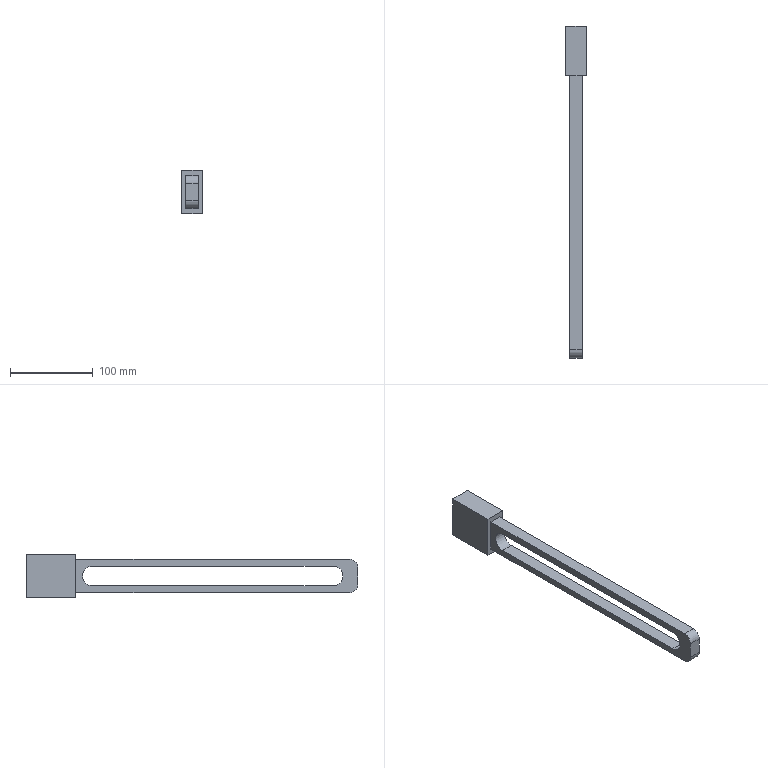Component | SolidWorks | TelescopicRod-1 | 1 solid | 17 faces | box 25 x 400 x 53 mm | volume 171670 mm3 | plane 13 | cylinder 4 | commonest cylinder face diameters 20 x2 24 x2
build123d program:
from build123d import *

# Parameters (mm, degrees)
SKETCH2_W           = 25
SKETCH2_H           = 53
BOSS_EXTRUDE1_DEPTH = 60
SKETCH3_W           = 15
SKETCH3_H           = 40
BOSS_EXTRUDE2_DEPTH = 340
FILLET1_R           = 10
CUT_EXTRUDE1_DEPTH  = 20


with BuildPart() as part:
    # Sketch2 → Boss-Extrude1 (new body)
    with BuildSketch(Plane.XY):
        with Locations((-42.5, 129)):
            Rectangle(SKETCH2_W, SKETCH2_H)
    extrude(amount=BOSS_EXTRUDE1_DEPTH)

    # Sketch3 → Boss-Extrude2 (add)
    with BuildSketch(Plane.XY.offset(60)):
        with Locations((-42.5, 129)):
            Rectangle(SKETCH3_W, SKETCH3_H)
    extrude(amount=BOSS_EXTRUDE2_DEPTH)

    # Fillet1
    fillet1_edges = [part.edges().sort_by_distance(p)[0] for p in [
        (-42.5, 109, 400),
        (-42.5, 149, 400),
    ]]
    fillet(fillet1_edges, radius=FILLET1_R)

    # Sketch4 → Cut-Extrude1 (cut)
    with BuildSketch(Plane.ZY.offset(50)):
        with BuildLine():
            Line((370, 117), (80, 117))
            ThreePointArc((80, 117), (68, 129), (80, 141))
            Line((80, 141), (370, 141))
            ThreePointArc((370, 141), (382, 129), (370, 117))
        make_face()
    extrude(amount=-CUT_EXTRUDE1_DEPTH, mode=Mode.SUBTRACT)


solid = part.part

# Placed as in the assembly
solid = solid.moved(Location((-496.496, 273.496, 244.626), (90, 0, 0)))
STEP:
#1=COLOUR_RGB('',0.7922,0.8196,0.9333);
#2=FILL_AREA_STYLE_COLOUR('',#1);
#3=FILL_AREA_STYLE('',(#2));
#4=SURFACE_STYLE_FILL_AREA(#3);
#5=SURFACE_SIDE_STYLE('',(#4));
#6=SURFACE_STYLE_USAGE(.BOTH.,#5);
#7=PRESENTATION_STYLE_ASSIGNMENT((#6));
#8=CARTESIAN_POINT('',(-21.712,10.768,15.753));
#9=VERTEX_POINT('',#8);
#10=CARTESIAN_POINT('',(-21.712,10.768,13.666));
#11=VERTEX_POINT('',#10);
#12=CARTESIAN_POINT('',(-21.712,10.768,15.753));
#13=DIRECTION('',(-0.,-0.,-1.));
#14=VECTOR('',#13,39.37);
#15=LINE('',#12,#14);
#16=EDGE_CURVE('',#9,#11,#15,.T.);
#17=ORIENTED_EDGE('',*,*,#16,.T.);
#18=CARTESIAN_POINT('',(-21.712,8.405,13.666));
#19=VERTEX_POINT('',#18);
#20=CARTESIAN_POINT('',(-21.712,8.405,13.666));
#21=DIRECTION('',(0.,1.,-0.));
#22=VECTOR('',#21,39.37);
#23=LINE('',#20,#22);
#24=EDGE_CURVE('',#19,#11,#23,.T.);
#25=ORIENTED_EDGE('',*,*,#24,.F.);
#26=CARTESIAN_POINT('',(-21.712,8.405,15.753));
#27=VERTEX_POINT('',#26);
#28=CARTESIAN_POINT('',(-21.712,8.405,15.753));
#29=DIRECTION('',(-0.,-0.,-1.));
#30=VECTOR('',#29,39.37);
#31=LINE('',#28,#30);
#32=EDGE_CURVE('',#27,#19,#31,.T.);
#33=ORIENTED_EDGE('',*,*,#32,.F.);
#34=CARTESIAN_POINT('',(-21.712,8.405,15.753));
#35=DIRECTION('',(0.,1.,-0.));
#36=VECTOR('',#35,39.37);
#37=LINE('',#34,#36);
#38=EDGE_CURVE('',#27,#9,#37,.T.);
#39=ORIENTED_EDGE('',*,*,#38,.T.);
#40=EDGE_LOOP('',(#17,#25,#33,#39));
#41=FACE_OUTER_BOUND('',#40,.T.);
#42=CARTESIAN_POINT('',(-21.712,8.405,15.753));
#43=DIRECTION('',(1.,-0.,-0.));
#44=DIRECTION('',(0.,1.,-0.));
#45=AXIS2_PLACEMENT_3D('',#42,#43,#44);
#46=PLANE('',#45);
#47=ADVANCED_FACE('',(#41),#46,.F.);
#48=CARTESIAN_POINT('',(-20.728,10.768,13.666));
#49=VERTEX_POINT('',#48);
#50=CARTESIAN_POINT('',(-21.712,10.768,13.666));
#51=DIRECTION('',(1.,-0.,0.));
#52=VECTOR('',#51,39.37);
#53=LINE('',#50,#52);
#54=EDGE_CURVE('',#11,#49,#53,.T.);
#55=ORIENTED_EDGE('',*,*,#54,.T.);
#56=CARTESIAN_POINT('',(-20.728,8.405,13.666));
#57=VERTEX_POINT('',#56);
#58=CARTESIAN_POINT('',(-20.728,8.405,13.666));
#59=DIRECTION('',(0.,1.,-0.));
#60=VECTOR('',#59,39.37);
#61=LINE('',#58,#60);
#62=EDGE_CURVE('',#57,#49,#61,.T.);
#63=ORIENTED_EDGE('',*,*,#62,.F.);
#64=CARTESIAN_POINT('',(-21.712,8.405,13.666));
#65=DIRECTION('',(1.,-0.,0.));
#66=VECTOR('',#65,39.37);
#67=LINE('',#64,#66);
#68=EDGE_CURVE('',#19,#57,#67,.T.);
#69=ORIENTED_EDGE('',*,*,#68,.F.);
#70=ORIENTED_EDGE('',*,*,#24,.T.);
#71=EDGE_LOOP('',(#55,#63,#69,#70));
#72=FACE_OUTER_BOUND('',#71,.T.);
#73=CARTESIAN_POINT('',(-21.712,8.405,13.666));
#74=DIRECTION('',(-0.,0.,1.));
#75=DIRECTION('',(-1.,0.,-0.));
#76=AXIS2_PLACEMENT_3D('',#73,#74,#75);
#77=PLANE('',#76);
#78=ADVANCED_FACE('',(#72),#77,.F.);
#79=CARTESIAN_POINT('',(-20.728,10.768,15.753));
#80=VERTEX_POINT('',#79);
#81=CARTESIAN_POINT('',(-20.728,10.768,15.753));
#82=DIRECTION('',(0.,0.,1.));
#83=VECTOR('',#82,39.37);
#84=LINE('',#81,#83);
#85=EDGE_CURVE('',#49,#80,#84,.T.);
#86=ORIENTED_EDGE('',*,*,#85,.T.);
#87=CARTESIAN_POINT('',(-20.728,8.405,15.753));
#88=VERTEX_POINT('',#87);
#89=CARTESIAN_POINT('',(-20.728,8.405,15.753));
#90=DIRECTION('',(0.,1.,-0.));
#91=VECTOR('',#90,39.37);
#92=LINE('',#89,#91);
#93=EDGE_CURVE('',#88,#80,#92,.T.);
#94=ORIENTED_EDGE('',*,*,#93,.F.);
#95=CARTESIAN_POINT('',(-20.728,8.405,15.753));
#96=DIRECTION('',(0.,0.,1.));
#97=VECTOR('',#96,39.37);
#98=LINE('',#95,#97);
#99=EDGE_CURVE('',#57,#88,#98,.T.);
#100=ORIENTED_EDGE('',*,*,#99,.F.);
#101=ORIENTED_EDGE('',*,*,#62,.T.);
#102=EDGE_LOOP('',(#86,#94,#100,#101));
#103=FACE_OUTER_BOUND('',#102,.T.);
#104=CARTESIAN_POINT('',(-20.728,8.405,15.753));
#105=DIRECTION('',(-1.,0.,0.));
#106=DIRECTION('',(-0.,-0.,-1.));
#107=AXIS2_PLACEMENT_3D('',#104,#105,#106);
#108=PLANE('',#107);
#109=ADVANCED_FACE('',(#103),#108,.F.);
#110=CARTESIAN_POINT('',(-21.712,10.768,15.753));
#111=DIRECTION('',(-1.,0.,0.));
#112=VECTOR('',#111,39.37);
#113=LINE('',#110,#112);
#114=EDGE_CURVE('',#80,#9,#113,.T.);
#115=ORIENTED_EDGE('',*,*,#114,.T.);
#116=ORIENTED_EDGE('',*,*,#38,.F.);
#117=CARTESIAN_POINT('',(-21.712,8.405,15.753));
#118=DIRECTION('',(-1.,0.,0.));
#119=VECTOR('',#118,39.37);
#120=LINE('',#117,#119);
#121=EDGE_CURVE('',#88,#27,#120,.T.);
#122=ORIENTED_EDGE('',*,*,#121,.F.);
#123=ORIENTED_EDGE('',*,*,#93,.T.);
#124=EDGE_LOOP('',(#115,#116,#122,#123));
#125=FACE_OUTER_BOUND('',#124,.T.);
#126=CARTESIAN_POINT('',(-21.712,8.405,15.753));
#127=DIRECTION('',(-0.,-0.,-1.));
#128=DIRECTION('',(0.,1.,-0.));
#129=AXIS2_PLACEMENT_3D('',#126,#127,#128);
#130=PLANE('',#129);
#131=ADVANCED_FACE('',(#125),#130,.F.);
#132=CARTESIAN_POINT('',(-21.516,8.405,15.497));
#133=VERTEX_POINT('',#132);
#134=CARTESIAN_POINT('',(-21.516,8.405,13.922));
#135=VERTEX_POINT('',#134);
#136=CARTESIAN_POINT('',(-21.516,8.405,15.497));
#137=DIRECTION('',(0.,-0.,-1.));
#138=VECTOR('',#137,39.37);
#139=LINE('',#136,#138);
#140=EDGE_CURVE('',#133,#135,#139,.T.);
#141=ORIENTED_EDGE('',*,*,#140,.F.);
#142=CARTESIAN_POINT('',(-20.925,8.405,15.497));
#143=VERTEX_POINT('',#142);
#144=CARTESIAN_POINT('',(-21.516,8.405,15.497));
#145=DIRECTION('',(-1.,0.,0.));
#146=VECTOR('',#145,39.37);
#147=LINE('',#144,#146);
#148=EDGE_CURVE('',#143,#133,#147,.T.);
#149=ORIENTED_EDGE('',*,*,#148,.F.);
#150=CARTESIAN_POINT('',(-20.925,8.405,13.922));
#151=VERTEX_POINT('',#150);
#152=CARTESIAN_POINT('',(-20.925,8.405,15.497));
#153=DIRECTION('',(-0.,0.,1.));
#154=VECTOR('',#153,39.37);
#155=LINE('',#152,#154);
#156=EDGE_CURVE('',#151,#143,#155,.T.);
#157=ORIENTED_EDGE('',*,*,#156,.F.);
#158=CARTESIAN_POINT('',(-21.516,8.405,13.922));
#159=DIRECTION('',(1.,-0.,-0.));
#160=VECTOR('',#159,39.37);
#161=LINE('',#158,#160);
#162=EDGE_CURVE('',#135,#151,#161,.T.);
#163=ORIENTED_EDGE('',*,*,#162,.F.);
#164=EDGE_LOOP('',(#141,#149,#157,#163));
#165=FACE_BOUND('',#164,.T.);
#166=ORIENTED_EDGE('',*,*,#32,.T.);
#167=ORIENTED_EDGE('',*,*,#68,.T.);
#168=ORIENTED_EDGE('',*,*,#99,.T.);
#169=ORIENTED_EDGE('',*,*,#121,.T.);
#170=EDGE_LOOP('',(#166,#167,#168,#169));
#171=FACE_OUTER_BOUND('',#170,.T.);
#172=CARTESIAN_POINT('',(-19.547,8.405,9.631));
#173=DIRECTION('',(-0.,-1.,0.));
#174=DIRECTION('',(1.,-0.,-0.));
#175=AXIS2_PLACEMENT_3D('',#172,#173,#174);
#176=PLANE('',#175);
#177=ADVANCED_FACE('',(#165,#171),#176,.T.);
#178=ORIENTED_EDGE('',*,*,#16,.F.);
#179=ORIENTED_EDGE('',*,*,#114,.F.);
#180=ORIENTED_EDGE('',*,*,#85,.F.);
#181=ORIENTED_EDGE('',*,*,#54,.F.);
#182=EDGE_LOOP('',(#178,#179,#180,#181));
#183=FACE_OUTER_BOUND('',#182,.T.);
#184=CARTESIAN_POINT('',(-19.547,10.768,9.631));
#185=DIRECTION('',(-0.,-1.,0.));
#186=DIRECTION('',(1.,-0.,-0.));
#187=AXIS2_PLACEMENT_3D('',#184,#185,#186);
#188=PLANE('',#187);
#189=ADVANCED_FACE('',(#183),#188,.F.);
#190=CARTESIAN_POINT('',(-21.516,-3.799,15.182));
#191=VERTEX_POINT('',#190);
#192=CARTESIAN_POINT('',(-21.516,7.618,15.182));
#193=VERTEX_POINT('',#192);
#194=CARTESIAN_POINT('',(-21.516,-3.799,15.182));
#195=DIRECTION('',(0.,1.,-0.));
#196=VECTOR('',#195,39.37);
#197=LINE('',#194,#196);
#198=EDGE_CURVE('',#191,#193,#197,.T.);
#199=ORIENTED_EDGE('',*,*,#198,.F.);
#200=CARTESIAN_POINT('',(-21.516,-3.799,14.237));
#201=VERTEX_POINT('',#200);
#202=CARTESIAN_POINT('',(-21.516,-3.799,14.71));
#203=DIRECTION('',(-1.,0.,-0.));
#204=DIRECTION('',(0.,-0.,-1.));
#205=AXIS2_PLACEMENT_3D('',#202,#203,#204);
#206=CIRCLE('',#205,0.4724);
#207=EDGE_CURVE('',#201,#191,#206,.T.);
#208=ORIENTED_EDGE('',*,*,#207,.F.);
#209=CARTESIAN_POINT('',(-21.516,7.618,14.237));
#210=VERTEX_POINT('',#209);
#211=CARTESIAN_POINT('',(-21.516,-3.799,14.237));
#212=DIRECTION('',(-0.,-1.,0.));
#213=VECTOR('',#212,39.37);
#214=LINE('',#211,#213);
#215=EDGE_CURVE('',#210,#201,#214,.T.);
#216=ORIENTED_EDGE('',*,*,#215,.F.);
#217=CARTESIAN_POINT('',(-21.516,7.618,14.71));
#218=DIRECTION('',(-1.,0.,-0.));
#219=DIRECTION('',(0.,0.,-1.));
#220=AXIS2_PLACEMENT_3D('',#217,#218,#219);
#221=CIRCLE('',#220,0.4724);
#222=EDGE_CURVE('',#193,#210,#221,.T.);
#223=ORIENTED_EDGE('',*,*,#222,.F.);
#224=EDGE_LOOP('',(#199,#208,#216,#223));
#225=FACE_BOUND('',#224,.T.);
#226=CARTESIAN_POINT('',(-21.516,-4.98,15.103));
#227=VERTEX_POINT('',#226);
#228=CARTESIAN_POINT('',(-21.516,-4.98,14.316));
#229=VERTEX_POINT('',#228);
#230=CARTESIAN_POINT('',(-21.516,-4.98,15.497));
#231=DIRECTION('',(0.,-0.,-1.));
#232=VECTOR('',#231,39.37);
#233=LINE('',#230,#232);
#234=EDGE_CURVE('',#227,#229,#233,.T.);
#235=ORIENTED_EDGE('',*,*,#234,.F.);
#236=CARTESIAN_POINT('',(-21.516,-4.587,15.497));
#237=VERTEX_POINT('',#236);
#238=CARTESIAN_POINT('',(-21.516,-4.587,15.103));
#239=DIRECTION('',(-1.,0.,-0.));
#240=DIRECTION('',(0.,0.,1.));
#241=AXIS2_PLACEMENT_3D('',#238,#239,#240);
#242=CIRCLE('',#241,0.3937);
#243=EDGE_CURVE('',#227,#237,#242,.T.);
#244=ORIENTED_EDGE('',*,*,#243,.T.);
#245=CARTESIAN_POINT('',(-21.516,-4.98,15.497));
#246=DIRECTION('',(0.,1.,-0.));
#247=VECTOR('',#246,39.37);
#248=LINE('',#245,#247);
#249=EDGE_CURVE('',#237,#133,#248,.T.);
#250=ORIENTED_EDGE('',*,*,#249,.T.);
#251=ORIENTED_EDGE('',*,*,#140,.T.);
#252=CARTESIAN_POINT('',(-21.516,-4.587,13.922));
#253=VERTEX_POINT('',#252);
#254=CARTESIAN_POINT('',(-21.516,-4.98,13.922));
#255=DIRECTION('',(0.,1.,-0.));
#256=VECTOR('',#255,39.37);
#257=LINE('',#254,#256);
#258=EDGE_CURVE('',#253,#135,#257,.T.);
#259=ORIENTED_EDGE('',*,*,#258,.F.);
#260=CARTESIAN_POINT('',(-21.516,-4.587,14.316));
#261=DIRECTION('',(-1.,0.,-0.));
#262=DIRECTION('',(0.,0.,1.));
#263=AXIS2_PLACEMENT_3D('',#260,#261,#262);
#264=CIRCLE('',#263,0.3937);
#265=EDGE_CURVE('',#253,#229,#264,.T.);
#266=ORIENTED_EDGE('',*,*,#265,.T.);
#267=EDGE_LOOP('',(#235,#244,#250,#251,#259,#266));
#268=FACE_OUTER_BOUND('',#267,.T.);
#269=CARTESIAN_POINT('',(-21.516,-4.98,15.497));
#270=DIRECTION('',(1.,-0.,0.));
#271=DIRECTION('',(-0.,0.,1.));
#272=AXIS2_PLACEMENT_3D('',#269,#270,#271);
#273=PLANE('',#272);
#274=ADVANCED_FACE('',(#225,#268),#273,.F.);
#275=CARTESIAN_POINT('',(-20.925,-4.587,13.922));
#276=VERTEX_POINT('',#275);
#277=CARTESIAN_POINT('',(-20.925,-4.98,13.922));
#278=DIRECTION('',(0.,1.,-0.));
#279=VECTOR('',#278,39.37);
#280=LINE('',#277,#279);
#281=EDGE_CURVE('',#276,#151,#280,.T.);
#282=ORIENTED_EDGE('',*,*,#281,.F.);
#283=CARTESIAN_POINT('',(-21.516,-4.587,13.922));
#284=DIRECTION('',(-1.,0.,0.));
#285=VECTOR('',#284,39.37);
#286=LINE('',#283,#285);
#287=EDGE_CURVE('',#276,#253,#286,.T.);
#288=ORIENTED_EDGE('',*,*,#287,.T.);
#289=ORIENTED_EDGE('',*,*,#258,.T.);
#290=ORIENTED_EDGE('',*,*,#162,.T.);
#291=EDGE_LOOP('',(#282,#288,#289,#290));
#292=FACE_OUTER_BOUND('',#291,.T.);
#293=CARTESIAN_POINT('',(-21.516,-4.98,13.922));
#294=DIRECTION('',(0.,0.,1.));
#295=DIRECTION('',(-0.,-1.,0.));
#296=AXIS2_PLACEMENT_3D('',#293,#294,#295);
#297=PLANE('',#296);
#298=ADVANCED_FACE('',(#292),#297,.F.);
#299=CARTESIAN_POINT('',(-20.925,7.618,14.237));
#300=VERTEX_POINT('',#299);
#301=CARTESIAN_POINT('',(-20.925,-3.799,14.237));
#302=VERTEX_POINT('',#301);
#303=CARTESIAN_POINT('',(-20.925,-4.98,14.237));
#304=DIRECTION('',(-0.,-1.,0.));
#305=VECTOR('',#304,39.37);
#306=LINE('',#303,#305);
#307=EDGE_CURVE('',#300,#302,#306,.T.);
#308=ORIENTED_EDGE('',*,*,#307,.T.);
#309=CARTESIAN_POINT('',(-20.925,-3.799,15.182));
#310=VERTEX_POINT('',#309);
#311=CARTESIAN_POINT('',(-20.925,-3.799,14.71));
#312=DIRECTION('',(-1.,0.,-0.));
#313=DIRECTION('',(0.,-0.,-1.));
#314=AXIS2_PLACEMENT_3D('',#311,#312,#313);
#315=CIRCLE('',#314,0.4724);
#316=EDGE_CURVE('',#302,#310,#315,.T.);
#317=ORIENTED_EDGE('',*,*,#316,.T.);
#318=CARTESIAN_POINT('',(-20.925,7.618,15.182));
#319=VERTEX_POINT('',#318);
#320=CARTESIAN_POINT('',(-20.925,-4.98,15.182));
#321=DIRECTION('',(0.,1.,-0.));
#322=VECTOR('',#321,39.37);
#323=LINE('',#320,#322);
#324=EDGE_CURVE('',#310,#319,#323,.T.);
#325=ORIENTED_EDGE('',*,*,#324,.T.);
#326=CARTESIAN_POINT('',(-20.925,7.618,14.71));
#327=DIRECTION('',(-1.,0.,-0.));
#328=DIRECTION('',(0.,0.,-1.));
#329=AXIS2_PLACEMENT_3D('',#326,#327,#328);
#330=CIRCLE('',#329,0.4724);
#331=EDGE_CURVE('',#319,#300,#330,.T.);
#332=ORIENTED_EDGE('',*,*,#331,.T.);
#333=EDGE_LOOP('',(#308,#317,#325,#332));
#334=FACE_BOUND('',#333,.T.);
#335=CARTESIAN_POINT('',(-20.925,-4.587,15.497));
#336=VERTEX_POINT('',#335);
#337=CARTESIAN_POINT('',(-20.925,-4.98,15.497));
#338=DIRECTION('',(0.,1.,-0.));
#339=VECTOR('',#338,39.37);
#340=LINE('',#337,#339);
#341=EDGE_CURVE('',#336,#143,#340,.T.);
#342=ORIENTED_EDGE('',*,*,#341,.F.);
#343=CARTESIAN_POINT('',(-20.925,-4.98,15.103));
#344=VERTEX_POINT('',#343);
#345=CARTESIAN_POINT('',(-20.925,-4.587,15.103));
#346=DIRECTION('',(1.,-0.,0.));
#347=DIRECTION('',(0.,0.,-1.));
#348=AXIS2_PLACEMENT_3D('',#345,#346,#347);
#349=CIRCLE('',#348,0.3937);
#350=EDGE_CURVE('',#336,#344,#349,.T.);
#351=ORIENTED_EDGE('',*,*,#350,.T.);
#352=CARTESIAN_POINT('',(-20.925,-4.98,14.316));
#353=VERTEX_POINT('',#352);
#354=CARTESIAN_POINT('',(-20.925,-4.98,15.497));
#355=DIRECTION('',(-0.,0.,1.));
#356=VECTOR('',#355,39.37);
#357=LINE('',#354,#356);
#358=EDGE_CURVE('',#353,#344,#357,.T.);
#359=ORIENTED_EDGE('',*,*,#358,.F.);
#360=CARTESIAN_POINT('',(-20.925,-4.587,14.316));
#361=DIRECTION('',(1.,-0.,0.));
#362=DIRECTION('',(0.,-0.,-1.));
#363=AXIS2_PLACEMENT_3D('',#360,#361,#362);
#364=CIRCLE('',#363,0.3937);
#365=EDGE_CURVE('',#353,#276,#364,.T.);
#366=ORIENTED_EDGE('',*,*,#365,.T.);
#367=ORIENTED_EDGE('',*,*,#281,.T.);
#368=ORIENTED_EDGE('',*,*,#156,.T.);
#369=EDGE_LOOP('',(#342,#351,#359,#366,#367,#368));
#370=FACE_OUTER_BOUND('',#369,.T.);
#371=CARTESIAN_POINT('',(-20.925,-4.98,15.497));
#372=DIRECTION('',(-1.,0.,-0.));
#373=DIRECTION('',(0.,-0.,-1.));
#374=AXIS2_PLACEMENT_3D('',#371,#372,#373);
#375=PLANE('',#374);
#376=ADVANCED_FACE('',(#334,#370),#375,.F.);
#377=ORIENTED_EDGE('',*,*,#249,.F.);
#378=CARTESIAN_POINT('',(-20.925,-4.587,15.497));
#379=DIRECTION('',(1.,-0.,-0.));
#380=VECTOR('',#379,39.37);
#381=LINE('',#378,#380);
#382=EDGE_CURVE('',#237,#336,#381,.T.);
#383=ORIENTED_EDGE('',*,*,#382,.T.);
#384=ORIENTED_EDGE('',*,*,#341,.T.);
#385=ORIENTED_EDGE('',*,*,#148,.T.);
#386=EDGE_LOOP('',(#377,#383,#384,#385));
#387=FACE_OUTER_BOUND('',#386,.T.);
#388=CARTESIAN_POINT('',(-21.516,-4.98,15.497));
#389=DIRECTION('',(-0.,-0.,-1.));
#390=DIRECTION('',(0.,1.,-0.));
#391=AXIS2_PLACEMENT_3D('',#388,#389,#390);
#392=PLANE('',#391);
#393=ADVANCED_FACE('',(#387),#392,.F.);
#394=ORIENTED_EDGE('',*,*,#358,.T.);
#395=CARTESIAN_POINT('',(-21.516,-4.98,15.103));
#396=DIRECTION('',(-1.,0.,0.));
#397=VECTOR('',#396,39.37);
#398=LINE('',#395,#397);
#399=EDGE_CURVE('',#344,#227,#398,.T.);
#400=ORIENTED_EDGE('',*,*,#399,.T.);
#401=ORIENTED_EDGE('',*,*,#234,.T.);
#402=CARTESIAN_POINT('',(-20.925,-4.98,14.316));
#403=DIRECTION('',(1.,-0.,-0.));
#404=VECTOR('',#403,39.37);
#405=LINE('',#402,#404);
#406=EDGE_CURVE('',#229,#353,#405,.T.);
#407=ORIENTED_EDGE('',*,*,#406,.T.);
#408=EDGE_LOOP('',(#394,#400,#401,#407));
#409=FACE_OUTER_BOUND('',#408,.T.);
#410=CARTESIAN_POINT('',(-19.547,-4.98,9.631));
#411=DIRECTION('',(-0.,-1.,0.));
#412=DIRECTION('',(1.,-0.,-0.));
#413=AXIS2_PLACEMENT_3D('',#410,#411,#412);
#414=PLANE('',#413);
#415=ADVANCED_FACE('',(#409),#414,.T.);
#416=ORIENTED_EDGE('',*,*,#350,.F.);
#417=ORIENTED_EDGE('',*,*,#382,.F.);
#418=ORIENTED_EDGE('',*,*,#243,.F.);
#419=ORIENTED_EDGE('',*,*,#399,.F.);
#420=EDGE_LOOP('',(#416,#417,#418,#419));
#421=FACE_OUTER_BOUND('',#420,.T.);
#422=CARTESIAN_POINT('',(-19.547,-4.587,15.103));
#423=DIRECTION('',(1.,-0.,-0.));
#424=DIRECTION('',(0.,1.,0.));
#425=AXIS2_PLACEMENT_3D('',#422,#423,#424);
#426=CYLINDRICAL_SURFACE('',#425,0.3937);
#427=ADVANCED_FACE('',(#421),#426,.T.);
#428=ORIENTED_EDGE('',*,*,#265,.F.);
#429=ORIENTED_EDGE('',*,*,#287,.F.);
#430=ORIENTED_EDGE('',*,*,#365,.F.);
#431=ORIENTED_EDGE('',*,*,#406,.F.);
#432=EDGE_LOOP('',(#428,#429,#430,#431));
#433=FACE_OUTER_BOUND('',#432,.T.);
#434=CARTESIAN_POINT('',(-19.547,-4.587,14.316));
#435=DIRECTION('',(-1.,0.,0.));
#436=DIRECTION('',(0.,-1.,0.));
#437=AXIS2_PLACEMENT_3D('',#434,#435,#436);
#438=CYLINDRICAL_SURFACE('',#437,0.3937);
#439=ADVANCED_FACE('',(#433),#438,.T.);
#440=CARTESIAN_POINT('',(-20.728,-3.799,14.237));
#441=DIRECTION('',(-1.,0.,-0.));
#442=VECTOR('',#441,39.37);
#443=LINE('',#440,#442);
#444=EDGE_CURVE('',#302,#201,#443,.T.);
#445=ORIENTED_EDGE('',*,*,#444,.T.);
#446=ORIENTED_EDGE('',*,*,#207,.T.);
#447=CARTESIAN_POINT('',(-20.728,-3.799,15.182));
#448=DIRECTION('',(-1.,0.,-0.));
#449=VECTOR('',#448,39.37);
#450=LINE('',#447,#449);
#451=EDGE_CURVE('',#310,#191,#450,.T.);
#452=ORIENTED_EDGE('',*,*,#451,.F.);
#453=ORIENTED_EDGE('',*,*,#316,.F.);
#454=EDGE_LOOP('',(#445,#446,#452,#453));
#455=FACE_OUTER_BOUND('',#454,.T.);
#456=CARTESIAN_POINT('',(-20.728,-3.799,14.71));
#457=DIRECTION('',(-1.,0.,-0.));
#458=DIRECTION('',(0.,-0.,-1.));
#459=AXIS2_PLACEMENT_3D('',#456,#457,#458);
#460=CYLINDRICAL_SURFACE('',#459,0.4724);
#461=ADVANCED_FACE('',(#455),#460,.F.);
#462=CARTESIAN_POINT('',(-20.728,7.618,14.237));
#463=DIRECTION('',(-1.,0.,-0.));
#464=VECTOR('',#463,39.37);
#465=LINE('',#462,#464);
#466=EDGE_CURVE('',#300,#210,#465,.T.);
#467=ORIENTED_EDGE('',*,*,#466,.T.);
#468=ORIENTED_EDGE('',*,*,#215,.T.);
#469=ORIENTED_EDGE('',*,*,#444,.F.);
#470=ORIENTED_EDGE('',*,*,#307,.F.);
#471=EDGE_LOOP('',(#467,#468,#469,#470));
#472=FACE_OUTER_BOUND('',#471,.T.);
#473=CARTESIAN_POINT('',(-20.728,-3.799,14.237));
#474=DIRECTION('',(0.,-0.,-1.));
#475=DIRECTION('',(1.,-0.,0.));
#476=AXIS2_PLACEMENT_3D('',#473,#474,#475);
#477=PLANE('',#476);
#478=ADVANCED_FACE('',(#472),#477,.F.);
#479=CARTESIAN_POINT('',(-20.728,7.618,15.182));
#480=DIRECTION('',(-1.,0.,-0.));
#481=VECTOR('',#480,39.37);
#482=LINE('',#479,#481);
#483=EDGE_CURVE('',#319,#193,#482,.T.);
#484=ORIENTED_EDGE('',*,*,#483,.T.);
#485=ORIENTED_EDGE('',*,*,#222,.T.);
#486=ORIENTED_EDGE('',*,*,#466,.F.);
#487=ORIENTED_EDGE('',*,*,#331,.F.);
#488=EDGE_LOOP('',(#484,#485,#486,#487));
#489=FACE_OUTER_BOUND('',#488,.T.);
#490=CARTESIAN_POINT('',(-20.728,7.618,14.71));
#491=DIRECTION('',(-1.,0.,-0.));
#492=DIRECTION('',(0.,0.,-1.));
#493=AXIS2_PLACEMENT_3D('',#490,#491,#492);
#494=CYLINDRICAL_SURFACE('',#493,0.4724);
#495=ADVANCED_FACE('',(#489),#494,.F.);
#496=ORIENTED_EDGE('',*,*,#451,.T.);
#497=ORIENTED_EDGE('',*,*,#198,.T.);
#498=ORIENTED_EDGE('',*,*,#483,.F.);
#499=ORIENTED_EDGE('',*,*,#324,.F.);
#500=EDGE_LOOP('',(#496,#497,#498,#499));
#501=FACE_OUTER_BOUND('',#500,.T.);
#502=CARTESIAN_POINT('',(-20.728,-3.799,15.182));
#503=DIRECTION('',(-0.,0.,1.));
#504=DIRECTION('',(-1.,0.,-0.));
#505=AXIS2_PLACEMENT_3D('',#502,#503,#504);
#506=PLANE('',#505);
#507=ADVANCED_FACE('',(#501),#506,.F.);
#508=CLOSED_SHELL('',(#47,#78,#109,#131,#177,#189,#274,#298,#376,#393,#415,#427,#439,#461,#478,#495,#507));
#509=MANIFOLD_SOLID_BREP('',#508);
#510=STYLED_ITEM('',(#7),#509);
#511=PRESENTATION_LAYER_ASSIGNMENT('','',(#510));
#512=CARTESIAN_POINT('',(0.,0.,0.));
#513=DIRECTION('',(0.,0.,1.));
#514=DIRECTION('',(1.,0.,0.));
#515=AXIS2_PLACEMENT_3D('',#512,#513,#514);
#516=(LENGTH_UNIT()NAMED_UNIT(*)SI_UNIT($,.METRE.));
#517=LENGTH_MEASURE_WITH_UNIT(LENGTH_MEASURE(0.0254),#516);
#518=DIMENSIONAL_EXPONENTS(1.,0.,0.,0.,0.,0.,0.);
#519=(CONVERSION_BASED_UNIT('',#517)LENGTH_UNIT()NAMED_UNIT(#518));
#520=UNCERTAINTY_MEASURE_WITH_UNIT(LENGTH_MEASURE(0.00001),#519,'','');
#521=(NAMED_UNIT(*)PLANE_ANGLE_UNIT()SI_UNIT($,.RADIAN.));
#522=(NAMED_UNIT(*)SI_UNIT($,.STERADIAN.)SOLID_ANGLE_UNIT());
#523=(GEOMETRIC_REPRESENTATION_CONTEXT(3)GLOBAL_UNCERTAINTY_ASSIGNED_CONTEXT((#520))GLOBAL_UNIT_ASSIGNED_CONTEXT((#519,#521,#522))REPRESENTATION_CONTEXT('',''));
#524=ADVANCED_BREP_SHAPE_REPRESENTATION('',(#509,#515),#523);
#525=(LENGTH_UNIT()NAMED_UNIT(*)SI_UNIT($,.METRE.));
#526=LENGTH_MEASURE_WITH_UNIT(LENGTH_MEASURE(0.0254),#525);
#527=DIMENSIONAL_EXPONENTS(1.,0.,0.,0.,0.,0.,0.);
#528=(CONVERSION_BASED_UNIT('',#526)LENGTH_UNIT()NAMED_UNIT(#527));
#529=UNCERTAINTY_MEASURE_WITH_UNIT(LENGTH_MEASURE(0.00001),#528,'','');
#530=(NAMED_UNIT(*)PLANE_ANGLE_UNIT()SI_UNIT($,.RADIAN.));
#531=(NAMED_UNIT(*)SI_UNIT($,.STERADIAN.)SOLID_ANGLE_UNIT());
#532=(GEOMETRIC_REPRESENTATION_CONTEXT(3)GLOBAL_UNCERTAINTY_ASSIGNED_CONTEXT((#529))GLOBAL_UNIT_ASSIGNED_CONTEXT((#528,#530,#531))REPRESENTATION_CONTEXT('',''));
#533=MECHANICAL_DESIGN_GEOMETRIC_PRESENTATION_REPRESENTATION('',(#510),#532);